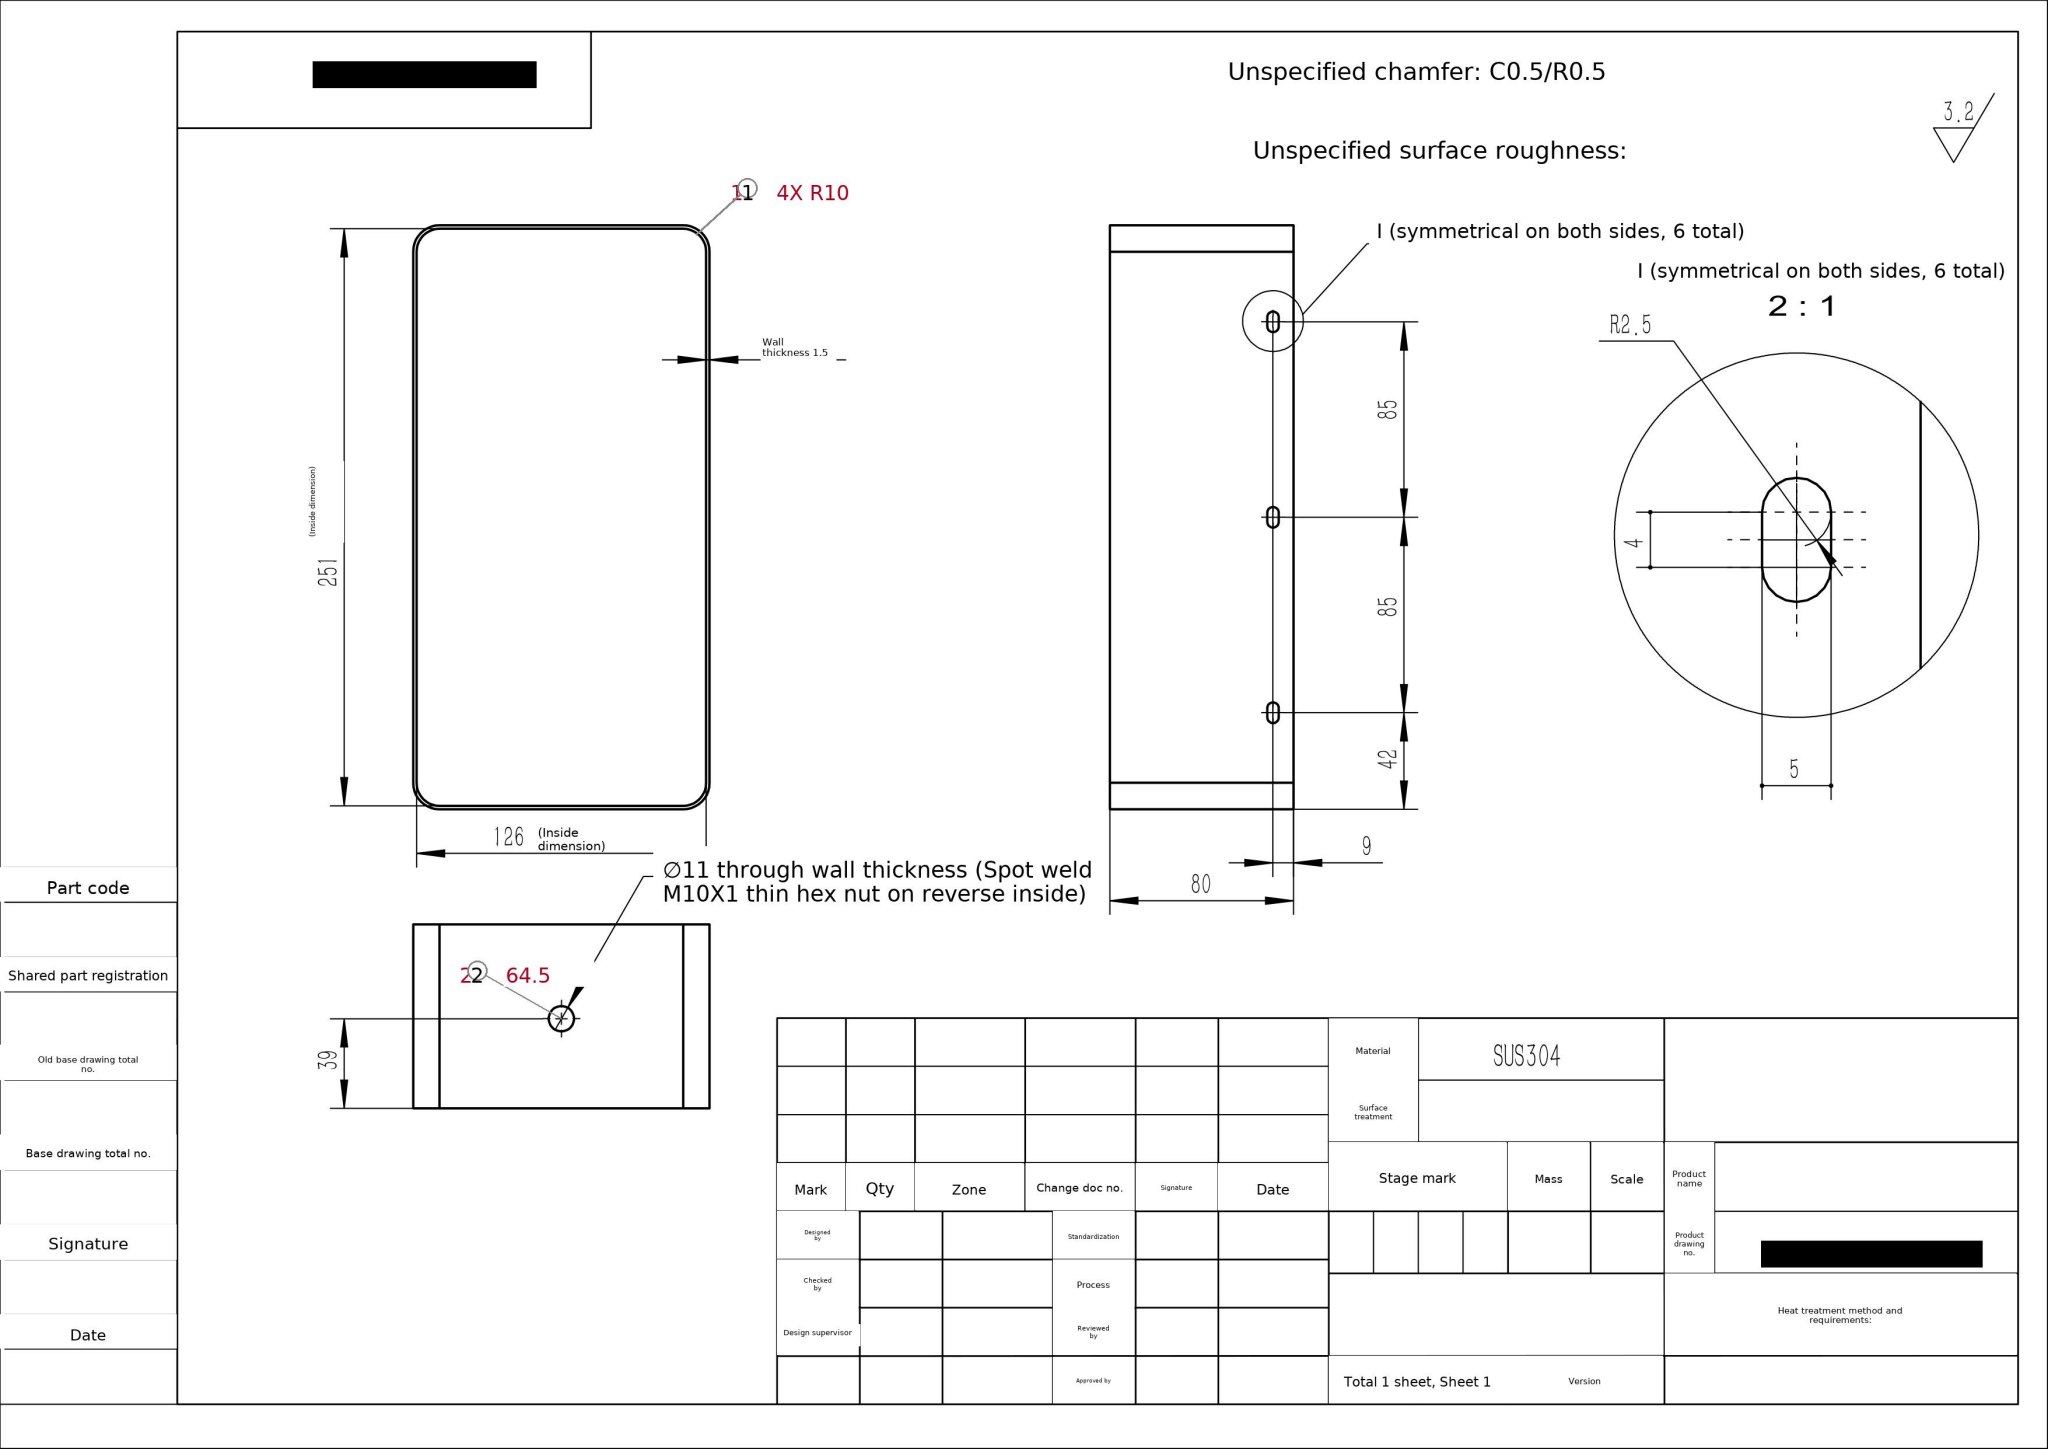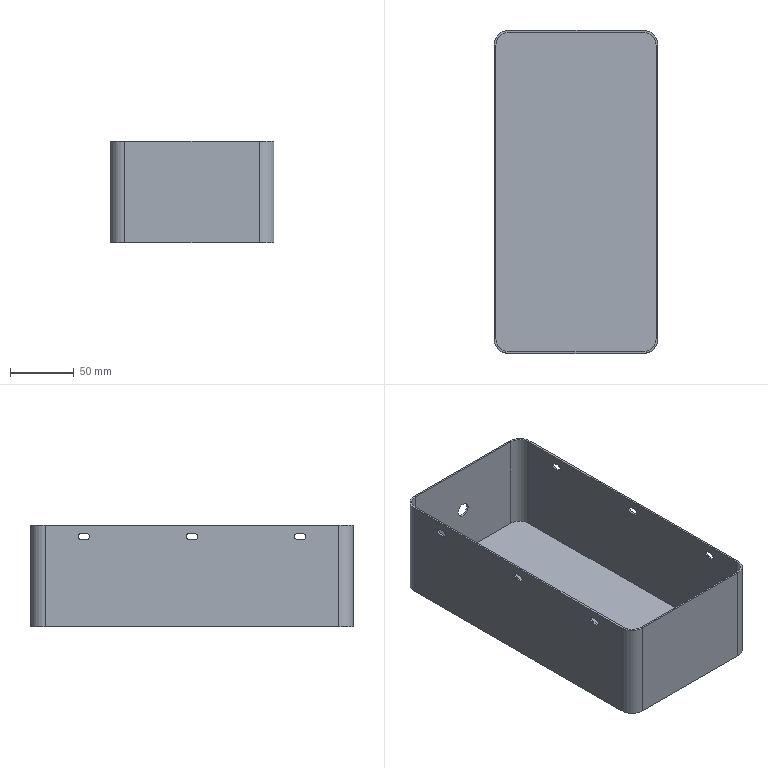Part | SolidWorks | mm | material SUS304 | 1 solid | 51 faces | box 129 x 254 x 80 mm | volume 135796 mm3 | cylinder 28 | plane 23 | commonest cylinder face diameters 5 x18 23 x4 20 x4 11 x2
build123d program:
from build123d import *

# Parameters (mm, degrees)
SKETCH1_W           = 129
SKETCH1_H           = 254
BOSS_EXTRUDE1_DEPTH = 80
FILLET1_R           = 11.5
SHELL1_T            = -1.5
SKETCH2_R           = 5.5
CUT_EXTRUDE1_DEPTH  = 10
CUT_EXTRUDE2_DEPTH  = 198.914


with BuildPart() as part:
    # Sketch1 → Boss-Extrude1 (new body)
    with BuildSketch(Plane.XY):
        Rectangle(SKETCH1_W, SKETCH1_H)
    extrude(amount=BOSS_EXTRUDE1_DEPTH)

    # Fillet1
    fillet1_edges = [part.edges().sort_by_distance(p)[0] for p in [
        (64.5, -127, 40),
        (-64.5, -127, 40),
        (-64.5, 127, 40),
        (64.5, 127, 40),
    ]]
    fillet(fillet1_edges, radius=FILLET1_R)

    # Shell1
    shell1_openings = [part.faces().sort_by_distance(p)[0] for p in [
        (0, 0, 80),
    ]]
    offset(amount=SHELL1_T, openings=shell1_openings, kind=Kind.INTERSECTION)

    # Sketch2 → Cut-Extrude1 (cut)
    with BuildSketch(Plane(origin=(0, 127, 0), x_dir=(1, 0, 0), z_dir=(0, 1, 0))):
        with Locations(Location((0, -41, 0), (0, 0, 270))):
            Circle(SKETCH2_R)
    extrude(amount=-CUT_EXTRUDE1_DEPTH, mode=Mode.SUBTRACT)

    # Sketch3 → Cut-Extrude2 (cut, through all)
    with BuildSketch(Plane.ZY.offset(64.5)):
        with BuildLine():
            Line((73.5, 87), (73.5, 83))
            ThreePointArc((73.5, 83), (71, 80.5), (68.5, 83))
            Line((68.5, 83), (68.5, 87))
            ThreePointArc((68.5, 87), (71, 89.5), (73.5, 87))
        make_face()
        with BuildLine():
            Line((73.5, 2), (73.5, -2))
            ThreePointArc((73.5, -2), (71, -4.5), (68.5, -2))
            Line((68.5, -2), (68.5, 2))
            ThreePointArc((68.5, 2), (71, 4.5), (73.5, 2))
        make_face()
        with BuildLine():
            Line((73.5, -83), (73.5, -87))
            ThreePointArc((73.5, -87), (71, -89.5), (68.5, -87))
            Line((68.5, -87), (68.5, -83))
            ThreePointArc((68.5, -83), (71, -80.5), (73.5, -83))
        make_face()
    extrude(amount=-CUT_EXTRUDE2_DEPTH, mode=Mode.SUBTRACT)


solid = part.part